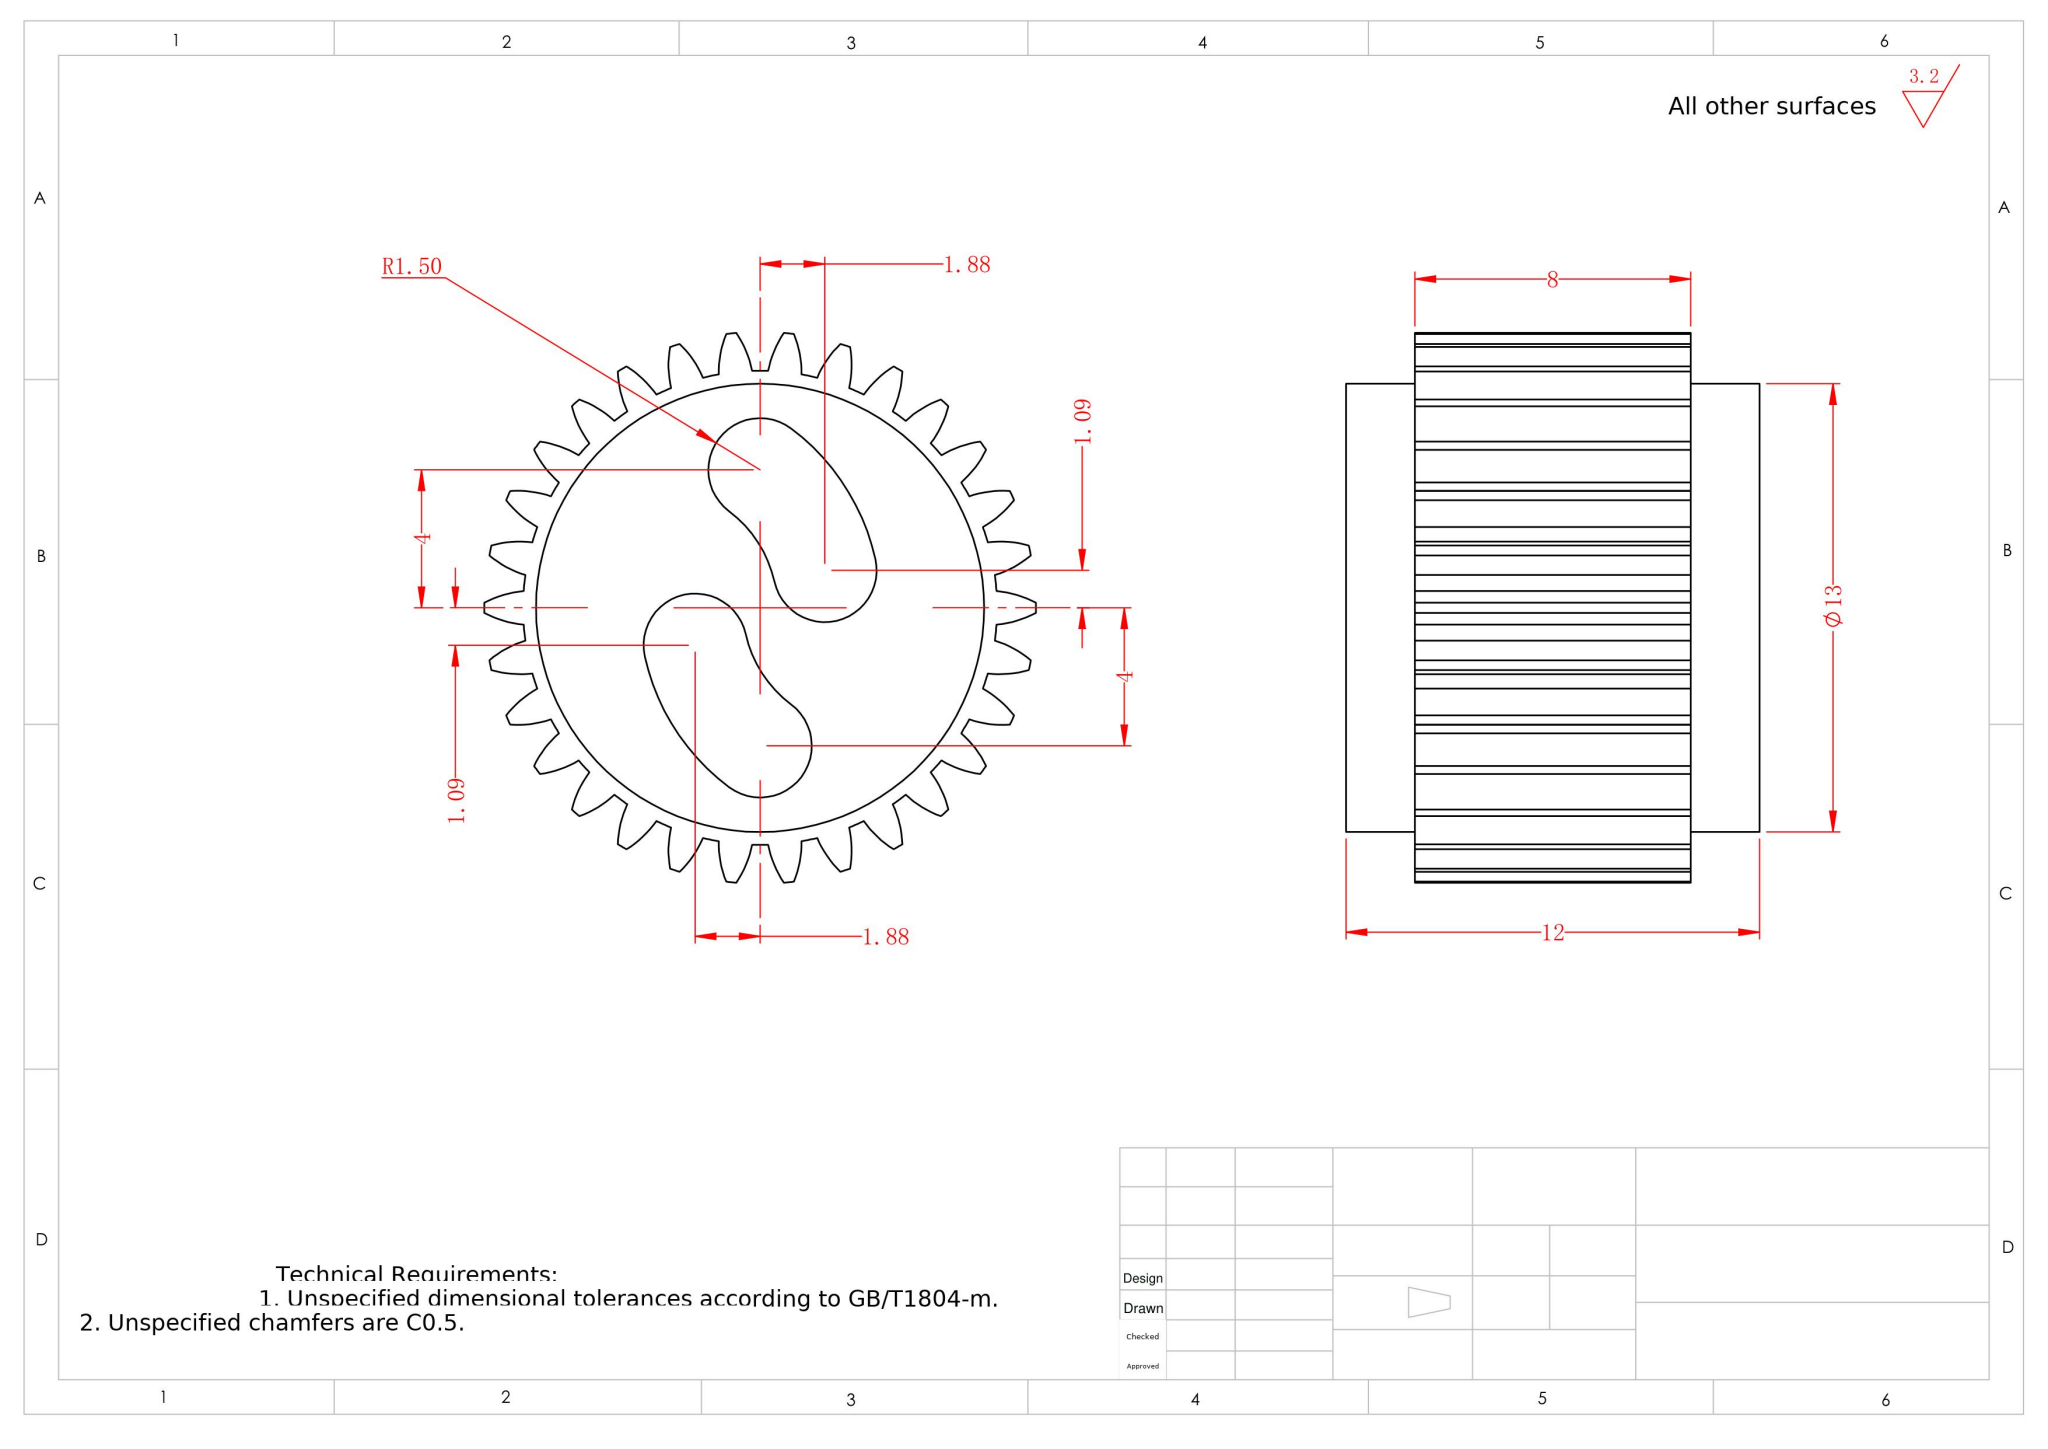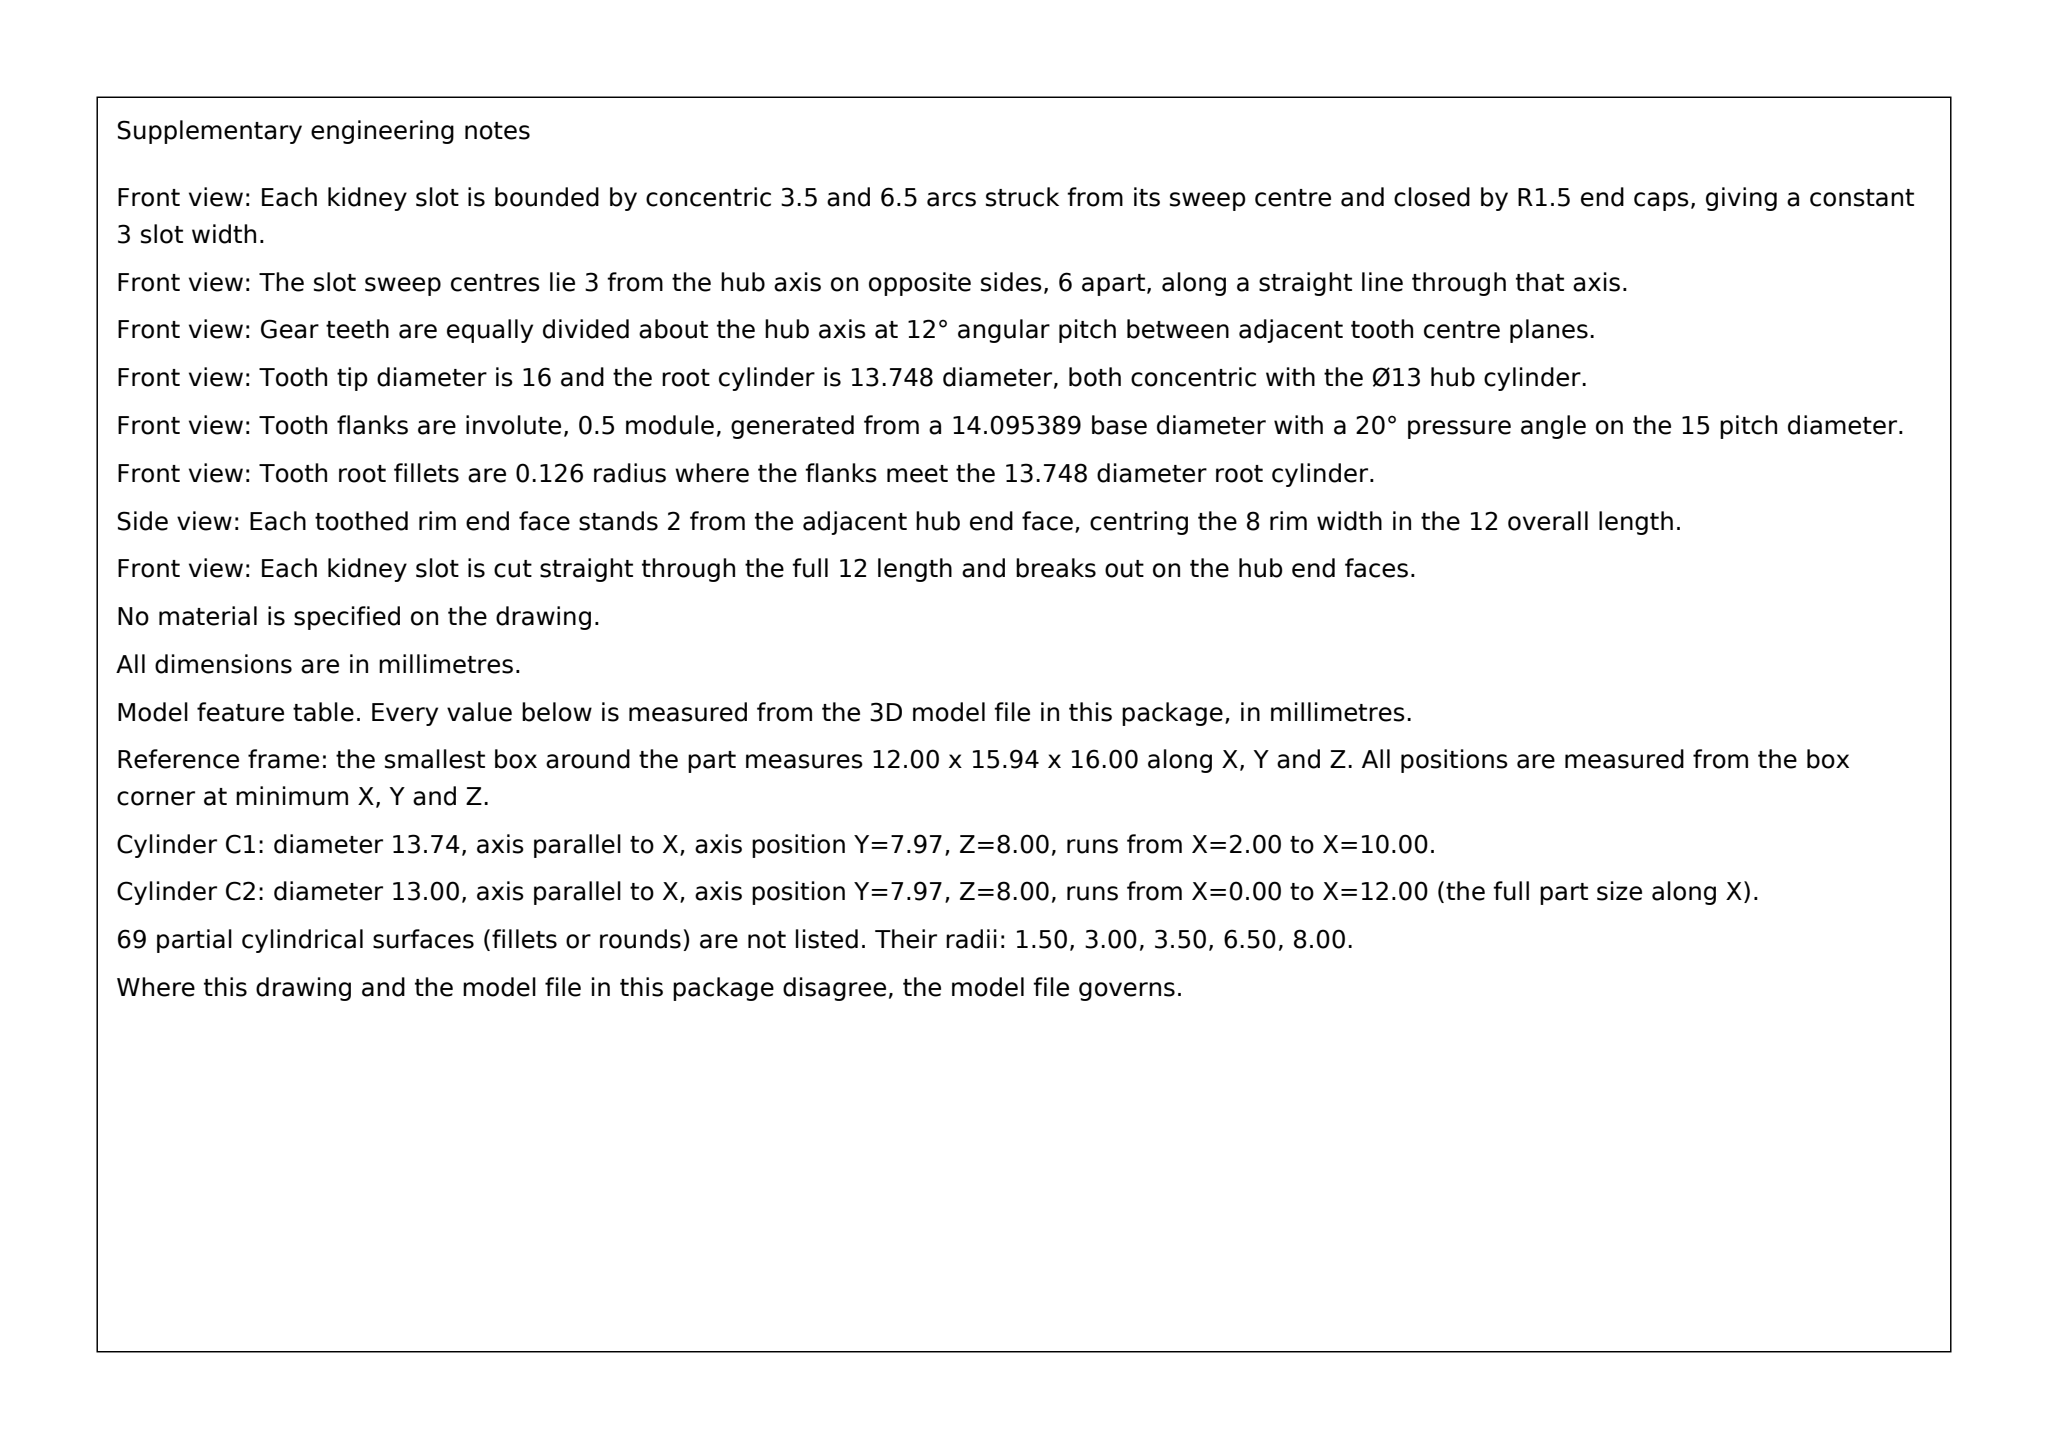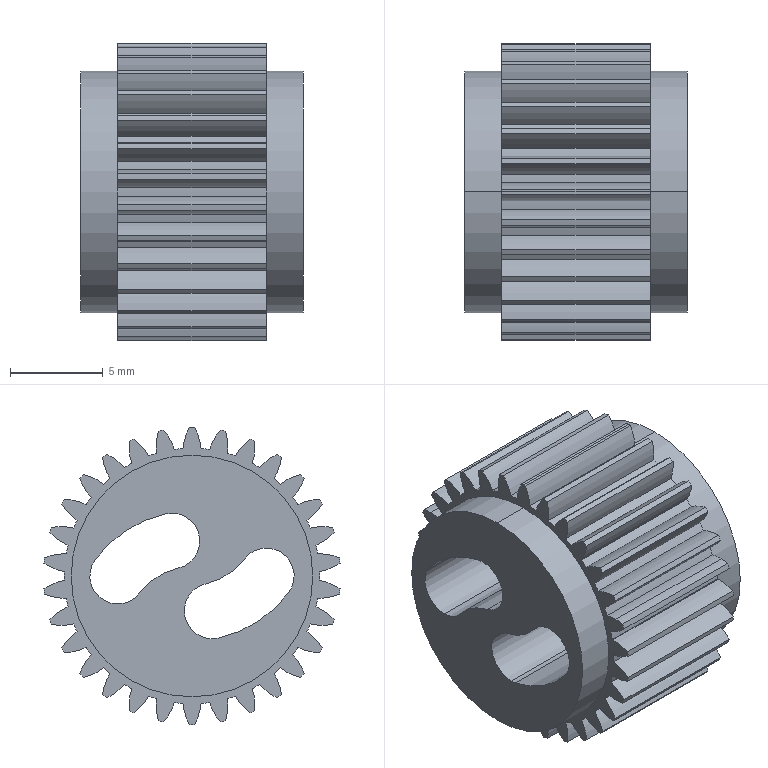Part | SolidWorks | mm | 1 solid | 143 faces | box 12 x 15.94 x 16 mm | volume 1487 mm3 | cylinder 139 | plane 4 | commonest cylinder face diameters 6 x64 16 x31 13.748 x30 13 x6 3 x6 7 x2
Drawing notes:
NO CENTRAL BORE - PART SOLID AT GEAR AXIS (DATUM A); CENTRE LINES FOR REFERENCE ONLY | from the solid: no cylinder listed on the gear axis (7.97, 8.0) other than the Ø13/Ø13.748/Ø16 outer surfaces
NO FILLETS OR CHAMFERS ON GEAR FACE / HUB TRANSITIONS - EDGES SHARP | from the solid: fillet_radii list empty and cones list empty
11. EACH KIDNEY SLOT IS BOUNDED BY ARCS R3.50 (INNER) AND R6.50 (OUTER), SLOT CENTRELINE R5.00, STRUCK FROM A CENTRE 3.00 FROM GEAR AXIS (DATUM A), THAT OFFSET BEING PERPENDICULAR TO THE RADIUS THROUGH THE 4.00 LOBE CENTRE AND DIRECTED AWAY FROM THE 1.09/1.88 LOBE | from the solid: cylinders dia 7.0 and dia 13.0, axis x, at (y7.97,z5.0) and (y7.97,z11.0), length 12 = 3.00 from gear axis (y7.97,z8.0); each is 5.00 from the dia 3.0 lobe cylinders of its slot
12. KIDNEY SLOT CLOCKING: THE R1.50 LOBE CENTRE AT 4.00 FROM GEAR AXIS (DATUM A) LIES ON A TOOTH CENTRELINE OF THE 30-TOOTH RIM; THE SECOND SLOT IS THE SAME FEATURE ROTATED 180° ABOUT DATUM A | from the solid: Gear axis is at (y,z)=(7.97,8.00); the 4.00 lobe centres are the dia 3.0 x 12 cylinders at (3.97,8.00) and (11.97,8.00), i.e. along ±y. The dia 6.0 x 8 tooth-flank arcs occur in mirror pairs straddling those directions ((0.93,7.66)/(0.93,8.34) and (15.01,7.66)/(15.01,8.34), ±2.77° about 180° and 0°, with further pairs at 12° steps), so a tooth, not a tooth space, is centred on the 4.00 lobe radius.
GEAR DATA: INVOLUTE SPUR, m=0.5, Z=30, PITCH Ø15, TIP Ø16 | from the solid: Tip cyl Ø16.0 x L8 (31 faces) with 30 tooth flank cyls Ø13.748; m=16/(30+2)=0.5, d=mz=15
ROOT Ø13.748, ADDENDUM 0.5, DEDENDUM 0.626, FACE WIDTH 8 | from the solid: Root cyl Ø13.748 x L8 count 30; gear face length 8.0 along x (planes x=2 to x=10)
build123d program:
from build123d import *

# Parameters (mm, degrees)
BASPROSKE_W         = 12
BASPROSKE_H         = 8
TOOTHCUT_DEPTH      = 17.492
TEETHCUTS_COUNT     = 30
BORSKE_R            = 0.4
BORE_DEPTH          = 50
CUT_EXTRUDE1_DEPTH  = 17.478
SKETCH2_R           = 10.638
SKETCH2_R_2         = 6.5
CUT_EXTRUDE2_DEPTH  = 2
CUT_EXTRUDE3_START  = -2
SKETCH3_R           = 10.295
SKETCH3_R_2         = 6.5
CUT_EXTRUDE3_DEPTH  = 2
SKETCH4_R           = 0.4
BOSS_EXTRUDE1_DEPTH = 12


with BuildPart() as part:
    # BasProSke → Base-Revolve (revolve)
    with BuildSketch(Plane(origin=(0, 0, 0), x_dir=(1, 0, 0), z_dir=(0, 1, 0)), mode=Mode.PRIVATE) as base_revolve_sk:
        with Locations((6, 4)):
            Rectangle(BASPROSKE_W, BASPROSKE_H)
    revolve(base_revolve_sk.sketch.rotate(Axis((-10, 0, 0), (1, 0, 0)), 180), axis=Axis((-10, 0, 0), (1, 0, 0)))

    # TooCutSke → ToothCut (cut, through all)
    with BuildSketch(Plane(origin=(0, 0, 0), x_dir=(0, 0, -1), z_dir=(1, 0, 0))):
        with BuildLine():
            ThreePointArc((0.2331, 6.87), (0, 6.874), (-0.2331, 6.87))
            ThreePointArc((-0.2331, 6.87), (-0.4123, 7.456), (-0.707, 7.994))
            ThreePointArc((-0.707, 7.994), (0, 8.025), (0.707, 7.994))
            ThreePointArc((0.707, 7.994), (0.4123, 7.456), (0.2331, 6.87))
        make_face()
    toothcut = extrude(amount=TOOTHCUT_DEPTH, mode=Mode.SUBTRACT)

    # TeethCuts: ToothCut ×30 about axis
    teethcuts_axis = Axis((0, 0, 0), (1, 0, 0))
    for i in range(1, TEETHCUTS_COUNT):
        add(toothcut.rotate(teethcuts_axis, i * 360 / TEETHCUTS_COUNT), mode=Mode.SUBTRACT)

    # BorSke → Bore (cut, symmetric)
    with BuildSketch(Plane(origin=(0, 0, 0), x_dir=(0, 0, -1), z_dir=(1, 0, 0))):
        with Locations(Location((0, 0, 0), (0, 0, 180))):
            Circle(BORSKE_R)
    extrude(amount=BORE_DEPTH, both=True, mode=Mode.SUBTRACT)

    # Sketch1 → Cut-Extrude1 (cut, through all)
    with BuildSketch(Plane(origin=(12, 0, 0), x_dir=(0, 0, -1), z_dir=(1, 0, 0))):
        with BuildLine():
            ThreePointArc((0.9, 2.8), (1.2, 4.9), (-0.9, 5.2))
            ThreePointArc((-0.9, 5.2), (-2.461, 3.525), (-3.345, 1.412))
            ThreePointArc((-3.345, 1.412), (-2.206, -0.3784), (-0.4165, 0.7601))
            ThreePointArc((-0.4165, 0.7601), (0.05922, 1.898), (0.9, 2.8))
        make_face()
        with BuildLine():
            ThreePointArc((3.345, -1.412), (2.206, 0.3784), (0.4165, -0.7601))
            ThreePointArc((0.4165, -0.7601), (-0.05922, -1.898), (-0.9, -2.8))
            ThreePointArc((-0.9, -2.8), (-1.2, -4.9), (0.9, -5.2))
            ThreePointArc((0.9, -5.2), (2.461, -3.525), (3.345, -1.412))
        make_face()
    extrude(amount=-CUT_EXTRUDE1_DEPTH, mode=Mode.SUBTRACT)

    # Sketch2 → Cut-Extrude2 (cut)
    with BuildSketch(Plane(origin=(12, 0, 0), x_dir=(0, 0, -1), z_dir=(1, 0, 0))):
        Circle(SKETCH2_R)
        Circle(SKETCH2_R_2, mode=Mode.SUBTRACT)
    extrude(amount=-CUT_EXTRUDE2_DEPTH, mode=Mode.SUBTRACT)

    # Sketch3 → Cut-Extrude3 (cut)
    with BuildSketch(Plane.ZY.offset(CUT_EXTRUDE3_START)):
        Circle(SKETCH3_R)
        with Locations(Location((0, 0, 0), (0, 0, 180))):
            Circle(SKETCH3_R_2, mode=Mode.SUBTRACT)
    extrude(amount=CUT_EXTRUDE3_DEPTH, mode=Mode.SUBTRACT)

    # Sketch4 → Boss-Extrude1 (add, through all)
    with BuildSketch(Plane(origin=(12, 0, 0), x_dir=(0, 0, -1), z_dir=(1, 0, 0))):
        Circle(SKETCH4_R)
    extrude(amount=-BOSS_EXTRUDE1_DEPTH)


solid = part.part